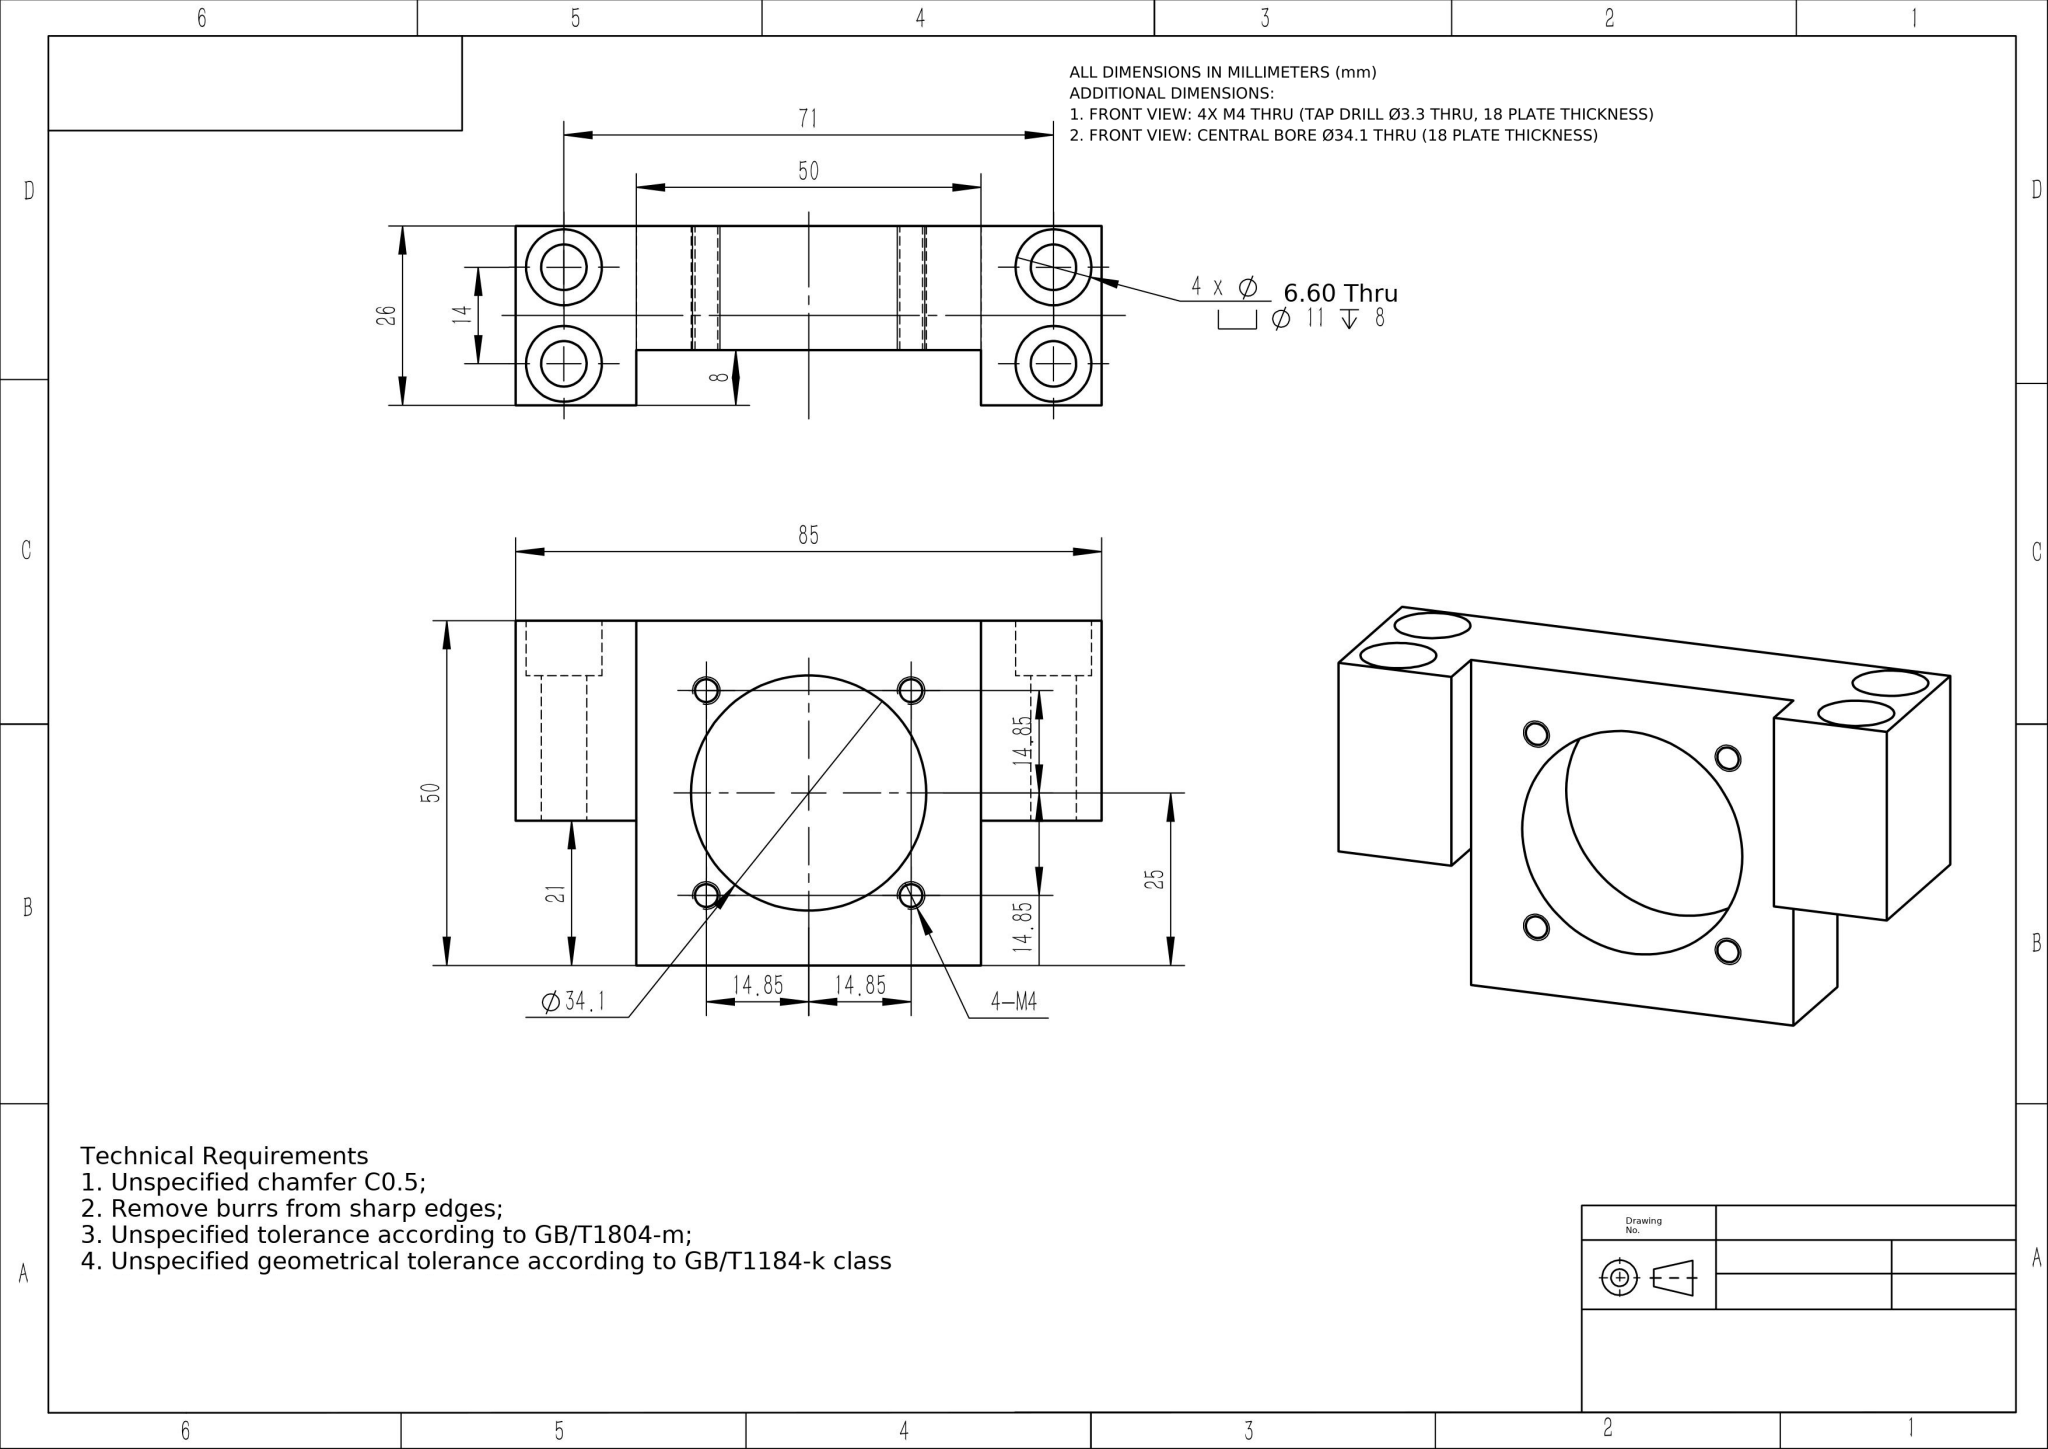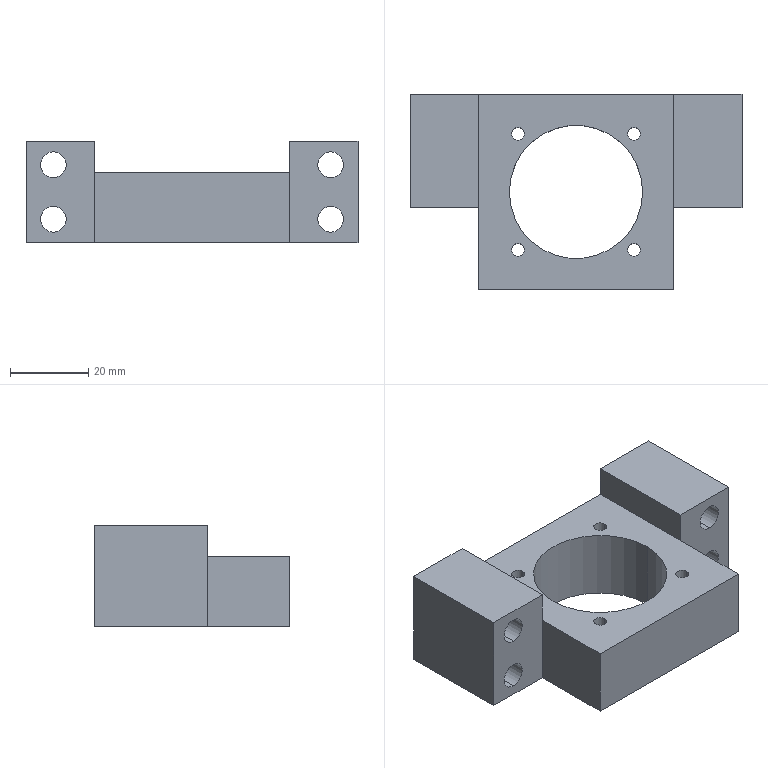Part | NX | mm | 1 solid | 44 faces | box 85 x 50 x 26 mm | volume 48420 mm3 | cylinder 26 | plane 18 | commonest cylinder face diameters 3.3 x8 11 x8 6.6 x8 34.1 x2